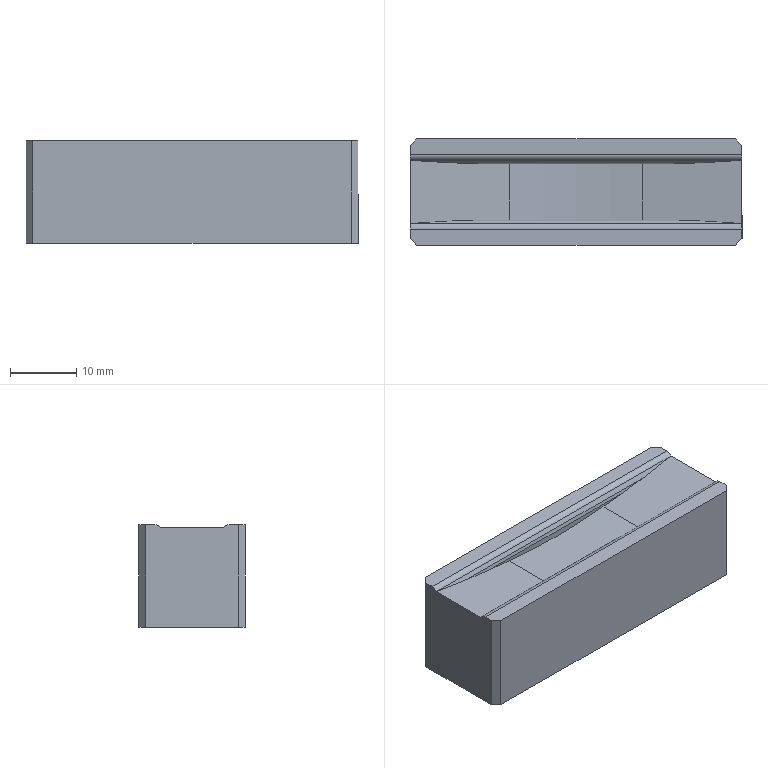Component | SolidWorks | 6.11-1937032105-0-1 | 1 solid | 40 faces | volume 10219 mm3 | plane 23 | cylinder 13 | cone 4 | commonest cylinder face diameters 5 x4 2 x4 6 x4 191.335 x1 | material 45#